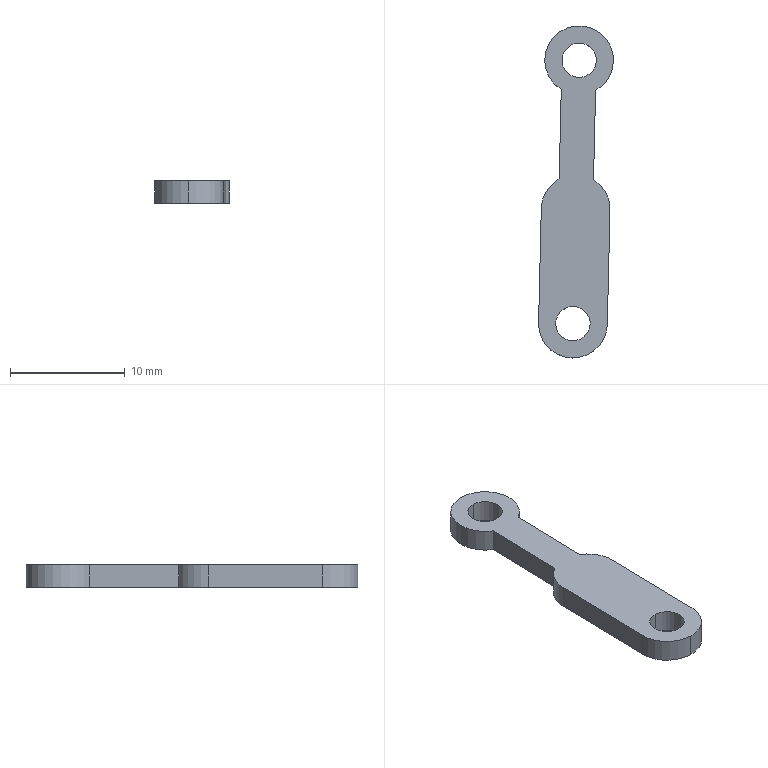Component | SolidWorks | 6-1 | 1 solid | 15 faces | box 6.54 x 28.99 x 2 mm | volume 248 mm3 | cylinder 9 | plane 6 | commonest cylinder face diameters 6 x5 3 x4
STEP:
#1=CARTESIAN_POINT('',(2.587,1.346,-1.179));
#2=VERTEX_POINT('',#1);
#3=CARTESIAN_POINT('',(2.59,1.464,-1.179));
#4=VERTEX_POINT('',#3);
#5=CARTESIAN_POINT('',(2.588,1.405,-1.179));
#6=DIRECTION('',(0.,0.,-1.));
#7=DIRECTION('',(0.02345,0.9997,0.));
#8=AXIS2_PLACEMENT_3D('',#5,#6,#7);
#9=CIRCLE('',#8,0.05906);
#10=EDGE_CURVE('',#2,#4,#9,.T.);
#11=ORIENTED_EDGE('',*,*,#10,.T.);
#12=CARTESIAN_POINT('',(2.59,1.464,-1.1));
#13=VERTEX_POINT('',#12);
#14=CARTESIAN_POINT('',(2.59,1.464,-1.179));
#15=DIRECTION('',(-0.,-0.,1.));
#16=VECTOR('',#15,39.37);
#17=LINE('',#14,#16);
#18=EDGE_CURVE('',#4,#13,#17,.T.);
#19=ORIENTED_EDGE('',*,*,#18,.T.);
#20=CARTESIAN_POINT('',(2.587,1.346,-1.1));
#21=VERTEX_POINT('',#20);
#22=CARTESIAN_POINT('',(2.588,1.405,-1.1));
#23=DIRECTION('',(0.,0.,-1.));
#24=DIRECTION('',(0.02345,0.9997,0.));
#25=AXIS2_PLACEMENT_3D('',#22,#23,#24);
#26=CIRCLE('',#25,0.05906);
#27=EDGE_CURVE('',#21,#13,#26,.T.);
#28=ORIENTED_EDGE('',*,*,#27,.F.);
#29=CARTESIAN_POINT('',(2.587,1.346,-1.179));
#30=DIRECTION('',(-0.,-0.,1.));
#31=VECTOR('',#30,39.37);
#32=LINE('',#29,#31);
#33=EDGE_CURVE('',#2,#21,#32,.T.);
#34=ORIENTED_EDGE('',*,*,#33,.F.);
#35=EDGE_LOOP('',(#11,#19,#28,#34));
#36=FACE_OUTER_BOUND('',#35,.T.);
#37=CARTESIAN_POINT('',(2.588,1.405,-1.179));
#38=DIRECTION('',(-0.,-0.,1.));
#39=DIRECTION('',(-0.02345,-0.9997,0.));
#40=AXIS2_PLACEMENT_3D('',#37,#38,#39);
#41=CYLINDRICAL_SURFACE('',#40,0.05906);
#42=ADVANCED_FACE('',(#36),#41,.F.);
#43=CARTESIAN_POINT('',(2.566,0.4406,-1.179));
#44=VERTEX_POINT('',#43);
#45=CARTESIAN_POINT('',(2.569,0.5587,-1.179));
#46=VERTEX_POINT('',#45);
#47=CARTESIAN_POINT('',(2.567,0.4997,-1.179));
#48=DIRECTION('',(0.,0.,-1.));
#49=DIRECTION('',(0.02345,0.9997,0.));
#50=AXIS2_PLACEMENT_3D('',#47,#48,#49);
#51=CIRCLE('',#50,0.05906);
#52=EDGE_CURVE('',#44,#46,#51,.T.);
#53=ORIENTED_EDGE('',*,*,#52,.T.);
#54=CARTESIAN_POINT('',(2.569,0.5587,-1.1));
#55=VERTEX_POINT('',#54);
#56=CARTESIAN_POINT('',(2.569,0.5587,-1.179));
#57=DIRECTION('',(-0.,-0.,1.));
#58=VECTOR('',#57,39.37);
#59=LINE('',#56,#58);
#60=EDGE_CURVE('',#46,#55,#59,.T.);
#61=ORIENTED_EDGE('',*,*,#60,.T.);
#62=CARTESIAN_POINT('',(2.566,0.4406,-1.1));
#63=VERTEX_POINT('',#62);
#64=CARTESIAN_POINT('',(2.567,0.4997,-1.1));
#65=DIRECTION('',(0.,0.,-1.));
#66=DIRECTION('',(0.02345,0.9997,0.));
#67=AXIS2_PLACEMENT_3D('',#64,#65,#66);
#68=CIRCLE('',#67,0.05906);
#69=EDGE_CURVE('',#63,#55,#68,.T.);
#70=ORIENTED_EDGE('',*,*,#69,.F.);
#71=CARTESIAN_POINT('',(2.566,0.4406,-1.179));
#72=DIRECTION('',(-0.,-0.,1.));
#73=VECTOR('',#72,39.37);
#74=LINE('',#71,#73);
#75=EDGE_CURVE('',#44,#63,#74,.T.);
#76=ORIENTED_EDGE('',*,*,#75,.F.);
#77=EDGE_LOOP('',(#53,#61,#70,#76));
#78=FACE_OUTER_BOUND('',#77,.T.);
#79=CARTESIAN_POINT('',(2.567,0.4997,-1.179));
#80=DIRECTION('',(-0.,-0.,1.));
#81=DIRECTION('',(-0.02345,-0.9997,0.));
#82=AXIS2_PLACEMENT_3D('',#79,#80,#81);
#83=CYLINDRICAL_SURFACE('',#82,0.05906);
#84=ADVANCED_FACE('',(#78),#83,.F.);
#85=CARTESIAN_POINT('',(2.564,0.3816,-1.179));
#86=VERTEX_POINT('',#85);
#87=CARTESIAN_POINT('',(2.449,0.5025,-1.179));
#88=VERTEX_POINT('',#87);
#89=CARTESIAN_POINT('',(2.567,0.4997,-1.179));
#90=DIRECTION('',(0.,0.,-1.));
#91=DIRECTION('',(0.02345,0.9997,0.));
#92=AXIS2_PLACEMENT_3D('',#89,#90,#91);
#93=CIRCLE('',#92,0.1181);
#94=EDGE_CURVE('',#86,#88,#93,.T.);
#95=ORIENTED_EDGE('',*,*,#94,.F.);
#96=CARTESIAN_POINT('',(2.564,0.3816,-1.1));
#97=VERTEX_POINT('',#96);
#98=CARTESIAN_POINT('',(2.564,0.3816,-1.179));
#99=DIRECTION('',(-0.,-0.,1.));
#100=VECTOR('',#99,39.37);
#101=LINE('',#98,#100);
#102=EDGE_CURVE('',#86,#97,#101,.T.);
#103=ORIENTED_EDGE('',*,*,#102,.T.);
#104=CARTESIAN_POINT('',(2.449,0.5025,-1.1));
#105=VERTEX_POINT('',#104);
#106=CARTESIAN_POINT('',(2.567,0.4997,-1.1));
#107=DIRECTION('',(0.,0.,-1.));
#108=DIRECTION('',(0.02345,0.9997,0.));
#109=AXIS2_PLACEMENT_3D('',#106,#107,#108);
#110=CIRCLE('',#109,0.1181);
#111=EDGE_CURVE('',#97,#105,#110,.T.);
#112=ORIENTED_EDGE('',*,*,#111,.T.);
#113=CARTESIAN_POINT('',(2.449,0.5025,-1.179));
#114=DIRECTION('',(-0.,-0.,1.));
#115=VECTOR('',#114,39.37);
#116=LINE('',#113,#115);
#117=EDGE_CURVE('',#88,#105,#116,.T.);
#118=ORIENTED_EDGE('',*,*,#117,.F.);
#119=EDGE_LOOP('',(#95,#103,#112,#118));
#120=FACE_OUTER_BOUND('',#119,.T.);
#121=CARTESIAN_POINT('',(2.567,0.4997,-1.179));
#122=DIRECTION('',(-0.,-0.,1.));
#123=DIRECTION('',(-0.02345,-0.9997,0.));
#124=AXIS2_PLACEMENT_3D('',#121,#122,#123);
#125=CYLINDRICAL_SURFACE('',#124,0.1181);
#126=ADVANCED_FACE('',(#120),#125,.T.);
#127=CARTESIAN_POINT('',(2.638,0.9942,-1.1));
#128=VERTEX_POINT('',#127);
#129=CARTESIAN_POINT('',(2.645,1.301,-1.1));
#130=VERTEX_POINT('',#129);
#131=CARTESIAN_POINT('',(2.648,1.404,-1.1));
#132=DIRECTION('',(0.02345,0.9997,0.));
#133=VECTOR('',#132,39.37);
#134=LINE('',#131,#133);
#135=EDGE_CURVE('',#128,#130,#134,.T.);
#136=ORIENTED_EDGE('',*,*,#135,.F.);
#137=CARTESIAN_POINT('',(2.638,0.9942,-1.179));
#138=VERTEX_POINT('',#137);
#139=CARTESIAN_POINT('',(2.638,0.9942,-1.179));
#140=DIRECTION('',(-0.,-0.,1.));
#141=VECTOR('',#140,39.37);
#142=LINE('',#139,#141);
#143=EDGE_CURVE('',#138,#128,#142,.T.);
#144=ORIENTED_EDGE('',*,*,#143,.F.);
#145=CARTESIAN_POINT('',(2.645,1.301,-1.179));
#146=VERTEX_POINT('',#145);
#147=CARTESIAN_POINT('',(2.648,1.404,-1.179));
#148=DIRECTION('',(0.02345,0.9997,0.));
#149=VECTOR('',#148,39.37);
#150=LINE('',#147,#149);
#151=EDGE_CURVE('',#138,#146,#150,.T.);
#152=ORIENTED_EDGE('',*,*,#151,.T.);
#153=CARTESIAN_POINT('',(2.645,1.301,-1.179));
#154=DIRECTION('',(-0.,-0.,1.));
#155=VECTOR('',#154,39.37);
#156=LINE('',#153,#155);
#157=EDGE_CURVE('',#146,#130,#156,.T.);
#158=ORIENTED_EDGE('',*,*,#157,.T.);
#159=EDGE_LOOP('',(#136,#144,#152,#158));
#160=FACE_OUTER_BOUND('',#159,.T.);
#161=CARTESIAN_POINT('',(2.648,1.404,-1.179));
#162=DIRECTION('',(0.9997,-0.02345,0.));
#163=DIRECTION('',(0.,0.,-1.));
#164=AXIS2_PLACEMENT_3D('',#161,#162,#163);
#165=PLANE('',#164);
#166=ADVANCED_FACE('',(#160),#165,.T.);
#167=CARTESIAN_POINT('',(2.695,0.8905,-1.1));
#168=VERTEX_POINT('',#167);
#169=CARTESIAN_POINT('',(2.576,0.8933,-1.1));
#170=DIRECTION('',(0.,0.,-1.));
#171=DIRECTION('',(0.02345,0.9997,0.));
#172=AXIS2_PLACEMENT_3D('',#169,#170,#171);
#173=CIRCLE('',#172,0.1181);
#174=EDGE_CURVE('',#128,#168,#173,.T.);
#175=ORIENTED_EDGE('',*,*,#174,.T.);
#176=CARTESIAN_POINT('',(2.695,0.8905,-1.179));
#177=VERTEX_POINT('',#176);
#178=CARTESIAN_POINT('',(2.695,0.8905,-1.179));
#179=DIRECTION('',(-0.,-0.,1.));
#180=VECTOR('',#179,39.37);
#181=LINE('',#178,#180);
#182=EDGE_CURVE('',#177,#168,#181,.T.);
#183=ORIENTED_EDGE('',*,*,#182,.F.);
#184=CARTESIAN_POINT('',(2.576,0.8933,-1.179));
#185=DIRECTION('',(0.,0.,-1.));
#186=DIRECTION('',(0.02345,0.9997,0.));
#187=AXIS2_PLACEMENT_3D('',#184,#185,#186);
#188=CIRCLE('',#187,0.1181);
#189=EDGE_CURVE('',#138,#177,#188,.T.);
#190=ORIENTED_EDGE('',*,*,#189,.F.);
#191=ORIENTED_EDGE('',*,*,#143,.T.);
#192=EDGE_LOOP('',(#175,#183,#190,#191));
#193=FACE_OUTER_BOUND('',#192,.T.);
#194=CARTESIAN_POINT('',(2.576,0.8933,-1.179));
#195=DIRECTION('',(-0.,-0.,1.));
#196=DIRECTION('',(-0.02345,-0.9997,0.));
#197=AXIS2_PLACEMENT_3D('',#194,#195,#196);
#198=CYLINDRICAL_SURFACE('',#197,0.1181);
#199=ADVANCED_FACE('',(#193),#198,.T.);
#200=CARTESIAN_POINT('',(2.685,0.4969,-1.1));
#201=VERTEX_POINT('',#200);
#202=CARTESIAN_POINT('',(2.707,1.402,-1.1));
#203=DIRECTION('',(0.02345,0.9997,0.));
#204=VECTOR('',#203,39.37);
#205=LINE('',#202,#204);
#206=EDGE_CURVE('',#201,#168,#205,.T.);
#207=ORIENTED_EDGE('',*,*,#206,.F.);
#208=CARTESIAN_POINT('',(2.685,0.4969,-1.179));
#209=VERTEX_POINT('',#208);
#210=CARTESIAN_POINT('',(2.685,0.4969,-1.179));
#211=DIRECTION('',(-0.,-0.,1.));
#212=VECTOR('',#211,39.37);
#213=LINE('',#210,#212);
#214=EDGE_CURVE('',#209,#201,#213,.T.);
#215=ORIENTED_EDGE('',*,*,#214,.F.);
#216=CARTESIAN_POINT('',(2.707,1.402,-1.179));
#217=DIRECTION('',(0.02345,0.9997,0.));
#218=VECTOR('',#217,39.37);
#219=LINE('',#216,#218);
#220=EDGE_CURVE('',#209,#177,#219,.T.);
#221=ORIENTED_EDGE('',*,*,#220,.T.);
#222=ORIENTED_EDGE('',*,*,#182,.T.);
#223=EDGE_LOOP('',(#207,#215,#221,#222));
#224=FACE_OUTER_BOUND('',#223,.T.);
#225=CARTESIAN_POINT('',(2.707,1.402,-1.179));
#226=DIRECTION('',(0.9997,-0.02345,0.));
#227=DIRECTION('',(0.,0.,-1.));
#228=AXIS2_PLACEMENT_3D('',#225,#226,#227);
#229=PLANE('',#228);
#230=ADVANCED_FACE('',(#224),#229,.T.);
#231=ORIENTED_EDGE('',*,*,#102,.F.);
#232=CARTESIAN_POINT('',(2.567,0.4997,-1.179));
#233=DIRECTION('',(0.,0.,-1.));
#234=DIRECTION('',(0.02345,0.9997,0.));
#235=AXIS2_PLACEMENT_3D('',#232,#233,#234);
#236=CIRCLE('',#235,0.1181);
#237=EDGE_CURVE('',#209,#86,#236,.T.);
#238=ORIENTED_EDGE('',*,*,#237,.F.);
#239=ORIENTED_EDGE('',*,*,#214,.T.);
#240=CARTESIAN_POINT('',(2.567,0.4997,-1.1));
#241=DIRECTION('',(0.,0.,-1.));
#242=DIRECTION('',(0.02345,0.9997,0.));
#243=AXIS2_PLACEMENT_3D('',#240,#241,#242);
#244=CIRCLE('',#243,0.1181);
#245=EDGE_CURVE('',#201,#97,#244,.T.);
#246=ORIENTED_EDGE('',*,*,#245,.T.);
#247=EDGE_LOOP('',(#231,#238,#239,#246));
#248=FACE_OUTER_BOUND('',#247,.T.);
#249=CARTESIAN_POINT('',(2.567,0.4997,-1.179));
#250=DIRECTION('',(-0.,-0.,1.));
#251=DIRECTION('',(-0.02345,-0.9997,0.));
#252=AXIS2_PLACEMENT_3D('',#249,#250,#251);
#253=CYLINDRICAL_SURFACE('',#252,0.1181);
#254=ADVANCED_FACE('',(#248),#253,.T.);
#255=CARTESIAN_POINT('',(2.458,0.8961,-1.1));
#256=VERTEX_POINT('',#255);
#257=CARTESIAN_POINT('',(2.47,1.408,-1.1));
#258=DIRECTION('',(0.02345,0.9997,0.));
#259=VECTOR('',#258,39.37);
#260=LINE('',#257,#259);
#261=EDGE_CURVE('',#105,#256,#260,.T.);
#262=ORIENTED_EDGE('',*,*,#261,.T.);
#263=CARTESIAN_POINT('',(2.458,0.8961,-1.179));
#264=VERTEX_POINT('',#263);
#265=CARTESIAN_POINT('',(2.458,0.8961,-1.179));
#266=DIRECTION('',(-0.,-0.,1.));
#267=VECTOR('',#266,39.37);
#268=LINE('',#265,#267);
#269=EDGE_CURVE('',#264,#256,#268,.T.);
#270=ORIENTED_EDGE('',*,*,#269,.F.);
#271=CARTESIAN_POINT('',(2.47,1.408,-1.179));
#272=DIRECTION('',(0.02345,0.9997,0.));
#273=VECTOR('',#272,39.37);
#274=LINE('',#271,#273);
#275=EDGE_CURVE('',#88,#264,#274,.T.);
#276=ORIENTED_EDGE('',*,*,#275,.F.);
#277=ORIENTED_EDGE('',*,*,#117,.T.);
#278=EDGE_LOOP('',(#262,#270,#276,#277));
#279=FACE_OUTER_BOUND('',#278,.T.);
#280=CARTESIAN_POINT('',(2.47,1.408,-1.179));
#281=DIRECTION('',(0.9997,-0.02345,0.));
#282=DIRECTION('',(0.,0.,-1.));
#283=AXIS2_PLACEMENT_3D('',#280,#281,#282);
#284=PLANE('',#283);
#285=ADVANCED_FACE('',(#279),#284,.F.);
#286=CARTESIAN_POINT('',(2.52,0.9969,-1.1));
#287=VERTEX_POINT('',#286);
#288=CARTESIAN_POINT('',(2.576,0.8933,-1.1));
#289=DIRECTION('',(0.,0.,-1.));
#290=DIRECTION('',(0.02345,0.9997,0.));
#291=AXIS2_PLACEMENT_3D('',#288,#289,#290);
#292=CIRCLE('',#291,0.1181);
#293=EDGE_CURVE('',#256,#287,#292,.T.);
#294=ORIENTED_EDGE('',*,*,#293,.T.);
#295=CARTESIAN_POINT('',(2.52,0.9969,-1.179));
#296=VERTEX_POINT('',#295);
#297=CARTESIAN_POINT('',(2.52,0.9969,-1.179));
#298=DIRECTION('',(-0.,-0.,1.));
#299=VECTOR('',#298,39.37);
#300=LINE('',#297,#299);
#301=EDGE_CURVE('',#296,#287,#300,.T.);
#302=ORIENTED_EDGE('',*,*,#301,.F.);
#303=CARTESIAN_POINT('',(2.576,0.8933,-1.179));
#304=DIRECTION('',(0.,0.,-1.));
#305=DIRECTION('',(0.02345,0.9997,0.));
#306=AXIS2_PLACEMENT_3D('',#303,#304,#305);
#307=CIRCLE('',#306,0.1181);
#308=EDGE_CURVE('',#264,#296,#307,.T.);
#309=ORIENTED_EDGE('',*,*,#308,.F.);
#310=ORIENTED_EDGE('',*,*,#269,.T.);
#311=EDGE_LOOP('',(#294,#302,#309,#310));
#312=FACE_OUTER_BOUND('',#311,.T.);
#313=CARTESIAN_POINT('',(2.576,0.8933,-1.179));
#314=DIRECTION('',(-0.,-0.,1.));
#315=DIRECTION('',(-0.02345,-0.9997,0.));
#316=AXIS2_PLACEMENT_3D('',#313,#314,#315);
#317=CYLINDRICAL_SURFACE('',#316,0.1181);
#318=ADVANCED_FACE('',(#312),#317,.T.);
#319=CARTESIAN_POINT('',(2.527,1.304,-1.1));
#320=VERTEX_POINT('',#319);
#321=CARTESIAN_POINT('',(2.529,1.406,-1.1));
#322=DIRECTION('',(0.02345,0.9997,0.));
#323=VECTOR('',#322,39.37);
#324=LINE('',#321,#323);
#325=EDGE_CURVE('',#287,#320,#324,.T.);
#326=ORIENTED_EDGE('',*,*,#325,.T.);
#327=CARTESIAN_POINT('',(2.527,1.304,-1.179));
#328=VERTEX_POINT('',#327);
#329=CARTESIAN_POINT('',(2.527,1.304,-1.179));
#330=DIRECTION('',(-0.,-0.,1.));
#331=VECTOR('',#330,39.37);
#332=LINE('',#329,#331);
#333=EDGE_CURVE('',#328,#320,#332,.T.);
#334=ORIENTED_EDGE('',*,*,#333,.F.);
#335=CARTESIAN_POINT('',(2.529,1.406,-1.179));
#336=DIRECTION('',(0.02345,0.9997,0.));
#337=VECTOR('',#336,39.37);
#338=LINE('',#335,#337);
#339=EDGE_CURVE('',#296,#328,#338,.T.);
#340=ORIENTED_EDGE('',*,*,#339,.F.);
#341=ORIENTED_EDGE('',*,*,#301,.T.);
#342=EDGE_LOOP('',(#326,#334,#340,#341));
#343=FACE_OUTER_BOUND('',#342,.T.);
#344=CARTESIAN_POINT('',(2.529,1.406,-1.179));
#345=DIRECTION('',(0.9997,-0.02345,0.));
#346=DIRECTION('',(0.,0.,-1.));
#347=AXIS2_PLACEMENT_3D('',#344,#345,#346);
#348=PLANE('',#347);
#349=ADVANCED_FACE('',(#343),#348,.F.);
#350=CARTESIAN_POINT('',(2.588,1.405,-1.1));
#351=DIRECTION('',(0.,0.,-1.));
#352=DIRECTION('',(0.02345,0.9997,0.));
#353=AXIS2_PLACEMENT_3D('',#350,#351,#352);
#354=CIRCLE('',#353,0.1181);
#355=EDGE_CURVE('',#320,#130,#354,.T.);
#356=ORIENTED_EDGE('',*,*,#355,.T.);
#357=ORIENTED_EDGE('',*,*,#157,.F.);
#358=CARTESIAN_POINT('',(2.588,1.405,-1.179));
#359=DIRECTION('',(0.,0.,-1.));
#360=DIRECTION('',(0.02345,0.9997,0.));
#361=AXIS2_PLACEMENT_3D('',#358,#359,#360);
#362=CIRCLE('',#361,0.1181);
#363=EDGE_CURVE('',#328,#146,#362,.T.);
#364=ORIENTED_EDGE('',*,*,#363,.F.);
#365=ORIENTED_EDGE('',*,*,#333,.T.);
#366=EDGE_LOOP('',(#356,#357,#364,#365));
#367=FACE_OUTER_BOUND('',#366,.T.);
#368=CARTESIAN_POINT('',(2.588,1.405,-1.179));
#369=DIRECTION('',(-0.,-0.,1.));
#370=DIRECTION('',(-0.02345,-0.9997,0.));
#371=AXIS2_PLACEMENT_3D('',#368,#369,#370);
#372=CYLINDRICAL_SURFACE('',#371,0.1181);
#373=ADVANCED_FACE('',(#367),#372,.T.);
#374=ORIENTED_EDGE('',*,*,#60,.F.);
#375=CARTESIAN_POINT('',(2.567,0.4997,-1.179));
#376=DIRECTION('',(0.,0.,-1.));
#377=DIRECTION('',(0.02345,0.9997,0.));
#378=AXIS2_PLACEMENT_3D('',#375,#376,#377);
#379=CIRCLE('',#378,0.05906);
#380=EDGE_CURVE('',#46,#44,#379,.T.);
#381=ORIENTED_EDGE('',*,*,#380,.T.);
#382=ORIENTED_EDGE('',*,*,#75,.T.);
#383=CARTESIAN_POINT('',(2.567,0.4997,-1.1));
#384=DIRECTION('',(0.,0.,-1.));
#385=DIRECTION('',(0.02345,0.9997,0.));
#386=AXIS2_PLACEMENT_3D('',#383,#384,#385);
#387=CIRCLE('',#386,0.05906);
#388=EDGE_CURVE('',#55,#63,#387,.T.);
#389=ORIENTED_EDGE('',*,*,#388,.F.);
#390=EDGE_LOOP('',(#374,#381,#382,#389));
#391=FACE_OUTER_BOUND('',#390,.T.);
#392=CARTESIAN_POINT('',(2.567,0.4997,-1.179));
#393=DIRECTION('',(-0.,-0.,1.));
#394=DIRECTION('',(-0.02345,-0.9997,0.));
#395=AXIS2_PLACEMENT_3D('',#392,#393,#394);
#396=CYLINDRICAL_SURFACE('',#395,0.05906);
#397=ADVANCED_FACE('',(#391),#396,.F.);
#398=ORIENTED_EDGE('',*,*,#18,.F.);
#399=CARTESIAN_POINT('',(2.588,1.405,-1.179));
#400=DIRECTION('',(0.,0.,-1.));
#401=DIRECTION('',(0.02345,0.9997,0.));
#402=AXIS2_PLACEMENT_3D('',#399,#400,#401);
#403=CIRCLE('',#402,0.05906);
#404=EDGE_CURVE('',#4,#2,#403,.T.);
#405=ORIENTED_EDGE('',*,*,#404,.T.);
#406=ORIENTED_EDGE('',*,*,#33,.T.);
#407=CARTESIAN_POINT('',(2.588,1.405,-1.1));
#408=DIRECTION('',(0.,0.,-1.));
#409=DIRECTION('',(0.02345,0.9997,0.));
#410=AXIS2_PLACEMENT_3D('',#407,#408,#409);
#411=CIRCLE('',#410,0.05906);
#412=EDGE_CURVE('',#13,#21,#411,.T.);
#413=ORIENTED_EDGE('',*,*,#412,.F.);
#414=EDGE_LOOP('',(#398,#405,#406,#413));
#415=FACE_OUTER_BOUND('',#414,.T.);
#416=CARTESIAN_POINT('',(2.588,1.405,-1.179));
#417=DIRECTION('',(-0.,-0.,1.));
#418=DIRECTION('',(-0.02345,-0.9997,0.));
#419=AXIS2_PLACEMENT_3D('',#416,#417,#418);
#420=CYLINDRICAL_SURFACE('',#419,0.05906);
#421=ADVANCED_FACE('',(#415),#420,.F.);
#422=ORIENTED_EDGE('',*,*,#52,.F.);
#423=ORIENTED_EDGE('',*,*,#380,.F.);
#424=EDGE_LOOP('',(#422,#423));
#425=FACE_BOUND('',#424,.T.);
#426=ORIENTED_EDGE('',*,*,#151,.F.);
#427=ORIENTED_EDGE('',*,*,#189,.T.);
#428=ORIENTED_EDGE('',*,*,#220,.F.);
#429=ORIENTED_EDGE('',*,*,#237,.T.);
#430=ORIENTED_EDGE('',*,*,#94,.T.);
#431=ORIENTED_EDGE('',*,*,#275,.T.);
#432=ORIENTED_EDGE('',*,*,#308,.T.);
#433=ORIENTED_EDGE('',*,*,#339,.T.);
#434=ORIENTED_EDGE('',*,*,#363,.T.);
#435=EDGE_LOOP('',(#426,#427,#428,#429,#430,#431,#432,#433,#434));
#436=FACE_OUTER_BOUND('',#435,.T.);
#437=ORIENTED_EDGE('',*,*,#10,.F.);
#438=ORIENTED_EDGE('',*,*,#404,.F.);
#439=EDGE_LOOP('',(#437,#438));
#440=FACE_BOUND('',#439,.T.);
#441=CARTESIAN_POINT('',(2.588,1.405,-1.179));
#442=DIRECTION('',(0.,0.,-1.));
#443=DIRECTION('',(0.02345,0.9997,0.));
#444=AXIS2_PLACEMENT_3D('',#441,#442,#443);
#445=PLANE('',#444);
#446=ADVANCED_FACE('',(#425,#436,#440),#445,.T.);
#447=ORIENTED_EDGE('',*,*,#69,.T.);
#448=ORIENTED_EDGE('',*,*,#388,.T.);
#449=EDGE_LOOP('',(#447,#448));
#450=FACE_BOUND('',#449,.T.);
#451=ORIENTED_EDGE('',*,*,#135,.T.);
#452=ORIENTED_EDGE('',*,*,#355,.F.);
#453=ORIENTED_EDGE('',*,*,#325,.F.);
#454=ORIENTED_EDGE('',*,*,#293,.F.);
#455=ORIENTED_EDGE('',*,*,#261,.F.);
#456=ORIENTED_EDGE('',*,*,#111,.F.);
#457=ORIENTED_EDGE('',*,*,#245,.F.);
#458=ORIENTED_EDGE('',*,*,#206,.T.);
#459=ORIENTED_EDGE('',*,*,#174,.F.);
#460=EDGE_LOOP('',(#451,#452,#453,#454,#455,#456,#457,#458,#459));
#461=FACE_OUTER_BOUND('',#460,.T.);
#462=ORIENTED_EDGE('',*,*,#27,.T.);
#463=ORIENTED_EDGE('',*,*,#412,.T.);
#464=EDGE_LOOP('',(#462,#463));
#465=FACE_BOUND('',#464,.T.);
#466=CARTESIAN_POINT('',(2.588,1.405,-1.1));
#467=DIRECTION('',(0.,0.,-1.));
#468=DIRECTION('',(0.02345,0.9997,0.));
#469=AXIS2_PLACEMENT_3D('',#466,#467,#468);
#470=PLANE('',#469);
#471=ADVANCED_FACE('',(#450,#461,#465),#470,.F.);
#472=CLOSED_SHELL('',(#42,#84,#126,#166,#199,#230,#254,#285,#318,#349,#373,#397,#421,#446,#471));
#473=MANIFOLD_SOLID_BREP('',#472);
#474=CARTESIAN_POINT('',(0.,0.,0.));
#475=DIRECTION('',(0.,0.,1.));
#476=DIRECTION('',(1.,0.,0.));
#477=AXIS2_PLACEMENT_3D('',#474,#475,#476);
#478=(LENGTH_UNIT()NAMED_UNIT(*)SI_UNIT($,.METRE.));
#479=LENGTH_MEASURE_WITH_UNIT(LENGTH_MEASURE(0.0254),#478);
#480=DIMENSIONAL_EXPONENTS(1.,0.,0.,0.,0.,0.,0.);
#481=(CONVERSION_BASED_UNIT('',#479)LENGTH_UNIT()NAMED_UNIT(#480));
#482=UNCERTAINTY_MEASURE_WITH_UNIT(LENGTH_MEASURE(0.00001),#481,'','');
#483=(NAMED_UNIT(*)PLANE_ANGLE_UNIT()SI_UNIT($,.RADIAN.));
#484=(NAMED_UNIT(*)SI_UNIT($,.STERADIAN.)SOLID_ANGLE_UNIT());
#485=(GEOMETRIC_REPRESENTATION_CONTEXT(3)GLOBAL_UNCERTAINTY_ASSIGNED_CONTEXT((#482))GLOBAL_UNIT_ASSIGNED_CONTEXT((#481,#483,#484))REPRESENTATION_CONTEXT('',''));
#486=ADVANCED_BREP_SHAPE_REPRESENTATION('',(#473,#477),#485);
#487=COLOUR_RGB('',0.7922,0.8196,0.9333);
#488=FILL_AREA_STYLE_COLOUR('',#487);
#489=FILL_AREA_STYLE('',(#488));
#490=SURFACE_STYLE_FILL_AREA(#489);
#491=SURFACE_SIDE_STYLE('',(#490));
#492=SURFACE_STYLE_USAGE(.BOTH.,#491);
#493=PRESENTATION_STYLE_ASSIGNMENT((#492));
#494=STYLED_ITEM('',(#493),#473);
#495=PRESENTATION_LAYER_ASSIGNMENT('','',(#494));
#496=(LENGTH_UNIT()NAMED_UNIT(*)SI_UNIT($,.METRE.));
#497=LENGTH_MEASURE_WITH_UNIT(LENGTH_MEASURE(0.0254),#496);
#498=DIMENSIONAL_EXPONENTS(1.,0.,0.,0.,0.,0.,0.);
#499=(CONVERSION_BASED_UNIT('',#497)LENGTH_UNIT()NAMED_UNIT(#498));
#500=UNCERTAINTY_MEASURE_WITH_UNIT(LENGTH_MEASURE(0.00001),#499,'','');
#501=(NAMED_UNIT(*)PLANE_ANGLE_UNIT()SI_UNIT($,.RADIAN.));
#502=(NAMED_UNIT(*)SI_UNIT($,.STERADIAN.)SOLID_ANGLE_UNIT());
#503=(GEOMETRIC_REPRESENTATION_CONTEXT(3)GLOBAL_UNCERTAINTY_ASSIGNED_CONTEXT((#500))GLOBAL_UNIT_ASSIGNED_CONTEXT((#499,#501,#502))REPRESENTATION_CONTEXT('',''));
#504=MECHANICAL_DESIGN_GEOMETRIC_PRESENTATION_REPRESENTATION('',(#494),#503);